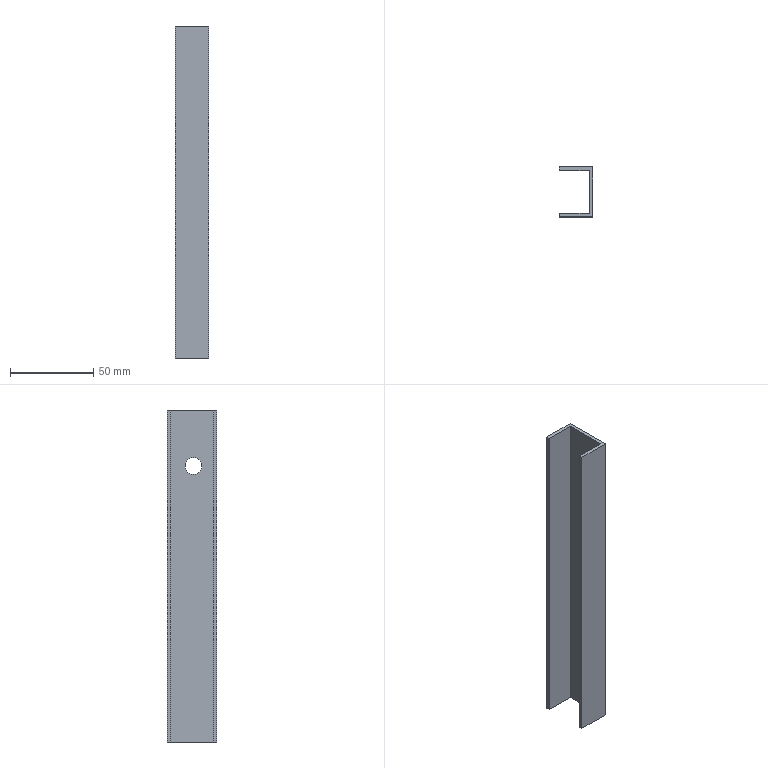Component | SolidWorks | Copy_of_Part3-10 | 1 solid | 12 faces | box 20 x 30 x 200 mm | volume 26243 mm3 | plane 10 | cylinder 2 | commonest cylinder face diameters 10 x2
build123d program:
from build123d import *

# Parameters (mm, degrees)
EXTRUDE_THIN1_DEPTH  = 200
SKETCH3_R            = 5
CUT_EXTRUDE1_2_DEPTH = 10


with BuildPart() as part:
    # Sketch1_2 → Extrude-Thin1 (new body)
    with BuildSketch(Plane.XY):
        Polygon((-20, 15.876), (0, 15.876), (0, -14.124), (-20, -14.124), (-20, -12.124), (-2, -12.124), (-2, 13.876), (-20, 13.876), align=None)
    extrude(amount=EXTRUDE_THIN1_DEPTH)

    # Sketch3 → Cut-Extrude1_2 (cut)
    with BuildSketch(Plane(origin=(0, 0, 0), x_dir=(0, 0, -1), z_dir=(1, 0, 0))):
        with Locations((-166.281, 0)):
            Circle(SKETCH3_R)
    extrude(amount=-CUT_EXTRUDE1_2_DEPTH, mode=Mode.SUBTRACT)


solid = part.part

# Placed as in the assembly
solid = solid.moved(Location((152, 214.124, -1266.092), (0, 0, 0)))
STEP:
#1=COLOUR_RGB('',0.7922,0.8196,0.9333);
#2=FILL_AREA_STYLE_COLOUR('',#1);
#3=FILL_AREA_STYLE('',(#2));
#4=SURFACE_STYLE_FILL_AREA(#3);
#5=SURFACE_SIDE_STYLE('',(#4));
#6=SURFACE_STYLE_USAGE(.BOTH.,#5);
#7=PRESENTATION_STYLE_ASSIGNMENT((#6));
#8=CARTESIAN_POINT('',(5.906,8.43,-43.103));
#9=VERTEX_POINT('',#8);
#10=CARTESIAN_POINT('',(5.906,8.43,-43.496));
#11=VERTEX_POINT('',#10);
#12=CARTESIAN_POINT('',(5.906,8.43,-43.3));
#13=DIRECTION('',(1.,0.,0.));
#14=DIRECTION('',(0.,0.,-1.));
#15=AXIS2_PLACEMENT_3D('',#12,#13,#14);
#16=CIRCLE('',#15,0.1969);
#17=EDGE_CURVE('',#9,#11,#16,.T.);
#18=ORIENTED_EDGE('',*,*,#17,.F.);
#19=CARTESIAN_POINT('',(5.984,8.43,-43.103));
#20=VERTEX_POINT('',#19);
#21=CARTESIAN_POINT('',(5.591,8.43,-43.103));
#22=DIRECTION('',(1.,0.,0.));
#23=VECTOR('',#22,39.37);
#24=LINE('',#21,#23);
#25=EDGE_CURVE('',#9,#20,#24,.T.);
#26=ORIENTED_EDGE('',*,*,#25,.T.);
#27=CARTESIAN_POINT('',(5.984,8.43,-43.496));
#28=VERTEX_POINT('',#27);
#29=CARTESIAN_POINT('',(5.984,8.43,-43.3));
#30=DIRECTION('',(1.,0.,0.));
#31=DIRECTION('',(0.,0.,-1.));
#32=AXIS2_PLACEMENT_3D('',#29,#30,#31);
#33=CIRCLE('',#32,0.1969);
#34=EDGE_CURVE('',#20,#28,#33,.T.);
#35=ORIENTED_EDGE('',*,*,#34,.T.);
#36=CARTESIAN_POINT('',(5.591,8.43,-43.496));
#37=DIRECTION('',(1.,0.,0.));
#38=VECTOR('',#37,39.37);
#39=LINE('',#36,#38);
#40=EDGE_CURVE('',#11,#28,#39,.T.);
#41=ORIENTED_EDGE('',*,*,#40,.F.);
#42=EDGE_LOOP('',(#18,#26,#35,#41));
#43=FACE_OUTER_BOUND('',#42,.T.);
#44=CARTESIAN_POINT('',(5.591,8.43,-43.3));
#45=DIRECTION('',(1.,0.,0.));
#46=DIRECTION('',(0.,0.,-1.));
#47=AXIS2_PLACEMENT_3D('',#44,#45,#46);
#48=CYLINDRICAL_SURFACE('',#47,0.1969);
#49=ADVANCED_FACE('',(#43),#48,.F.);
#50=CARTESIAN_POINT('',(5.906,7.953,-49.846));
#51=VERTEX_POINT('',#50);
#52=CARTESIAN_POINT('',(5.197,7.953,-49.846));
#53=VERTEX_POINT('',#52);
#54=CARTESIAN_POINT('',(5.984,7.953,-49.846));
#55=DIRECTION('',(-1.,-0.,0.));
#56=VECTOR('',#55,39.37);
#57=LINE('',#54,#56);
#58=EDGE_CURVE('',#51,#53,#57,.T.);
#59=ORIENTED_EDGE('',*,*,#58,.T.);
#60=CARTESIAN_POINT('',(5.197,7.953,-41.972));
#61=VERTEX_POINT('',#60);
#62=CARTESIAN_POINT('',(5.197,7.953,-41.972));
#63=DIRECTION('',(0.,0.,-1.));
#64=VECTOR('',#63,39.37);
#65=LINE('',#62,#64);
#66=EDGE_CURVE('',#61,#53,#65,.T.);
#67=ORIENTED_EDGE('',*,*,#66,.F.);
#68=CARTESIAN_POINT('',(5.906,7.953,-41.972));
#69=VERTEX_POINT('',#68);
#70=CARTESIAN_POINT('',(5.984,7.953,-41.972));
#71=DIRECTION('',(-1.,-0.,0.));
#72=VECTOR('',#71,39.37);
#73=LINE('',#70,#72);
#74=EDGE_CURVE('',#69,#61,#73,.T.);
#75=ORIENTED_EDGE('',*,*,#74,.F.);
#76=CARTESIAN_POINT('',(5.906,7.953,-41.972));
#77=DIRECTION('',(0.,0.,-1.));
#78=VECTOR('',#77,39.37);
#79=LINE('',#76,#78);
#80=EDGE_CURVE('',#69,#51,#79,.T.);
#81=ORIENTED_EDGE('',*,*,#80,.T.);
#82=EDGE_LOOP('',(#59,#67,#75,#81));
#83=FACE_OUTER_BOUND('',#82,.T.);
#84=CARTESIAN_POINT('',(5.984,7.953,-41.972));
#85=DIRECTION('',(0.,-1.,0.));
#86=DIRECTION('',(1.,0.,0.));
#87=AXIS2_PLACEMENT_3D('',#84,#85,#86);
#88=PLANE('',#87);
#89=ADVANCED_FACE('',(#83),#88,.F.);
#90=CARTESIAN_POINT('',(5.197,7.874,-49.846));
#91=VERTEX_POINT('',#90);
#92=CARTESIAN_POINT('',(5.197,7.874,-49.846));
#93=DIRECTION('',(0.,1.,0.));
#94=VECTOR('',#93,39.37);
#95=LINE('',#92,#94);
#96=EDGE_CURVE('',#91,#53,#95,.T.);
#97=ORIENTED_EDGE('',*,*,#96,.F.);
#98=CARTESIAN_POINT('',(5.197,7.874,-41.972));
#99=VERTEX_POINT('',#98);
#100=CARTESIAN_POINT('',(5.197,7.874,-41.972));
#101=DIRECTION('',(0.,0.,-1.));
#102=VECTOR('',#101,39.37);
#103=LINE('',#100,#102);
#104=EDGE_CURVE('',#99,#91,#103,.T.);
#105=ORIENTED_EDGE('',*,*,#104,.F.);
#106=CARTESIAN_POINT('',(5.197,7.874,-41.972));
#107=DIRECTION('',(0.,1.,0.));
#108=VECTOR('',#107,39.37);
#109=LINE('',#106,#108);
#110=EDGE_CURVE('',#99,#61,#109,.T.);
#111=ORIENTED_EDGE('',*,*,#110,.T.);
#112=ORIENTED_EDGE('',*,*,#66,.T.);
#113=EDGE_LOOP('',(#97,#105,#111,#112));
#114=FACE_OUTER_BOUND('',#113,.T.);
#115=CARTESIAN_POINT('',(5.197,7.874,-41.972));
#116=DIRECTION('',(-1.,0.,0.));
#117=DIRECTION('',(0.,0.,1.));
#118=AXIS2_PLACEMENT_3D('',#115,#116,#117);
#119=PLANE('',#118);
#120=ADVANCED_FACE('',(#114),#119,.T.);
#121=CARTESIAN_POINT('',(5.984,7.874,-49.846));
#122=VERTEX_POINT('',#121);
#123=CARTESIAN_POINT('',(5.984,7.874,-49.846));
#124=DIRECTION('',(-1.,-0.,0.));
#125=VECTOR('',#124,39.37);
#126=LINE('',#123,#125);
#127=EDGE_CURVE('',#122,#91,#126,.T.);
#128=ORIENTED_EDGE('',*,*,#127,.F.);
#129=CARTESIAN_POINT('',(5.984,7.874,-41.972));
#130=VERTEX_POINT('',#129);
#131=CARTESIAN_POINT('',(5.984,7.874,-41.972));
#132=DIRECTION('',(0.,0.,-1.));
#133=VECTOR('',#132,39.37);
#134=LINE('',#131,#133);
#135=EDGE_CURVE('',#130,#122,#134,.T.);
#136=ORIENTED_EDGE('',*,*,#135,.F.);
#137=CARTESIAN_POINT('',(5.984,7.874,-41.972));
#138=DIRECTION('',(-1.,-0.,0.));
#139=VECTOR('',#138,39.37);
#140=LINE('',#137,#139);
#141=EDGE_CURVE('',#130,#99,#140,.T.);
#142=ORIENTED_EDGE('',*,*,#141,.T.);
#143=ORIENTED_EDGE('',*,*,#104,.T.);
#144=EDGE_LOOP('',(#128,#136,#142,#143));
#145=FACE_OUTER_BOUND('',#144,.T.);
#146=CARTESIAN_POINT('',(5.984,7.874,-41.972));
#147=DIRECTION('',(0.,-1.,0.));
#148=DIRECTION('',(1.,0.,0.));
#149=AXIS2_PLACEMENT_3D('',#146,#147,#148);
#150=PLANE('',#149);
#151=ADVANCED_FACE('',(#145),#150,.T.);
#152=CARTESIAN_POINT('',(5.984,8.43,-43.3));
#153=DIRECTION('',(1.,0.,0.));
#154=DIRECTION('',(0.,0.,-1.));
#155=AXIS2_PLACEMENT_3D('',#152,#153,#154);
#156=CIRCLE('',#155,0.1969);
#157=EDGE_CURVE('',#28,#20,#156,.T.);
#158=ORIENTED_EDGE('',*,*,#157,.F.);
#159=ORIENTED_EDGE('',*,*,#34,.F.);
#160=EDGE_LOOP('',(#158,#159));
#161=FACE_BOUND('',#160,.T.);
#162=CARTESIAN_POINT('',(5.984,9.055,-49.846));
#163=VERTEX_POINT('',#162);
#164=CARTESIAN_POINT('',(5.984,7.874,-49.846));
#165=DIRECTION('',(0.,-1.,0.));
#166=VECTOR('',#165,39.37);
#167=LINE('',#164,#166);
#168=EDGE_CURVE('',#163,#122,#167,.T.);
#169=ORIENTED_EDGE('',*,*,#168,.F.);
#170=CARTESIAN_POINT('',(5.984,9.055,-41.972));
#171=VERTEX_POINT('',#170);
#172=CARTESIAN_POINT('',(5.984,9.055,-41.972));
#173=DIRECTION('',(0.,0.,-1.));
#174=VECTOR('',#173,39.37);
#175=LINE('',#172,#174);
#176=EDGE_CURVE('',#171,#163,#175,.T.);
#177=ORIENTED_EDGE('',*,*,#176,.F.);
#178=CARTESIAN_POINT('',(5.984,7.874,-41.972));
#179=DIRECTION('',(0.,-1.,0.));
#180=VECTOR('',#179,39.37);
#181=LINE('',#178,#180);
#182=EDGE_CURVE('',#171,#130,#181,.T.);
#183=ORIENTED_EDGE('',*,*,#182,.T.);
#184=ORIENTED_EDGE('',*,*,#135,.T.);
#185=EDGE_LOOP('',(#169,#177,#183,#184));
#186=FACE_OUTER_BOUND('',#185,.T.);
#187=CARTESIAN_POINT('',(5.984,7.874,-41.972));
#188=DIRECTION('',(1.,0.,0.));
#189=DIRECTION('',(0.,0.,-1.));
#190=AXIS2_PLACEMENT_3D('',#187,#188,#189);
#191=PLANE('',#190);
#192=ADVANCED_FACE('',(#161,#186),#191,.T.);
#193=CARTESIAN_POINT('',(5.197,9.055,-49.846));
#194=VERTEX_POINT('',#193);
#195=CARTESIAN_POINT('',(5.984,9.055,-49.846));
#196=DIRECTION('',(1.,0.,0.));
#197=VECTOR('',#196,39.37);
#198=LINE('',#195,#197);
#199=EDGE_CURVE('',#194,#163,#198,.T.);
#200=ORIENTED_EDGE('',*,*,#199,.F.);
#201=CARTESIAN_POINT('',(5.197,9.055,-41.972));
#202=VERTEX_POINT('',#201);
#203=CARTESIAN_POINT('',(5.197,9.055,-41.972));
#204=DIRECTION('',(0.,0.,-1.));
#205=VECTOR('',#204,39.37);
#206=LINE('',#203,#205);
#207=EDGE_CURVE('',#202,#194,#206,.T.);
#208=ORIENTED_EDGE('',*,*,#207,.F.);
#209=CARTESIAN_POINT('',(5.984,9.055,-41.972));
#210=DIRECTION('',(1.,0.,0.));
#211=VECTOR('',#210,39.37);
#212=LINE('',#209,#211);
#213=EDGE_CURVE('',#202,#171,#212,.T.);
#214=ORIENTED_EDGE('',*,*,#213,.T.);
#215=ORIENTED_EDGE('',*,*,#176,.T.);
#216=EDGE_LOOP('',(#200,#208,#214,#215));
#217=FACE_OUTER_BOUND('',#216,.T.);
#218=CARTESIAN_POINT('',(5.984,9.055,-41.972));
#219=DIRECTION('',(0.,1.,0.));
#220=DIRECTION('',(0.,0.,1.));
#221=AXIS2_PLACEMENT_3D('',#218,#219,#220);
#222=PLANE('',#221);
#223=ADVANCED_FACE('',(#217),#222,.T.);
#224=CARTESIAN_POINT('',(5.197,8.976,-49.846));
#225=VERTEX_POINT('',#224);
#226=CARTESIAN_POINT('',(5.197,8.976,-49.846));
#227=DIRECTION('',(0.,1.,0.));
#228=VECTOR('',#227,39.37);
#229=LINE('',#226,#228);
#230=EDGE_CURVE('',#225,#194,#229,.T.);
#231=ORIENTED_EDGE('',*,*,#230,.F.);
#232=CARTESIAN_POINT('',(5.197,8.976,-41.972));
#233=VERTEX_POINT('',#232);
#234=CARTESIAN_POINT('',(5.197,8.976,-41.972));
#235=DIRECTION('',(0.,0.,-1.));
#236=VECTOR('',#235,39.37);
#237=LINE('',#234,#236);
#238=EDGE_CURVE('',#233,#225,#237,.T.);
#239=ORIENTED_EDGE('',*,*,#238,.F.);
#240=CARTESIAN_POINT('',(5.197,8.976,-41.972));
#241=DIRECTION('',(0.,1.,0.));
#242=VECTOR('',#241,39.37);
#243=LINE('',#240,#242);
#244=EDGE_CURVE('',#233,#202,#243,.T.);
#245=ORIENTED_EDGE('',*,*,#244,.T.);
#246=ORIENTED_EDGE('',*,*,#207,.T.);
#247=EDGE_LOOP('',(#231,#239,#245,#246));
#248=FACE_OUTER_BOUND('',#247,.T.);
#249=CARTESIAN_POINT('',(5.197,8.976,-41.972));
#250=DIRECTION('',(-1.,0.,0.));
#251=DIRECTION('',(0.,0.,1.));
#252=AXIS2_PLACEMENT_3D('',#249,#250,#251);
#253=PLANE('',#252);
#254=ADVANCED_FACE('',(#248),#253,.T.);
#255=CARTESIAN_POINT('',(5.906,8.976,-49.846));
#256=VERTEX_POINT('',#255);
#257=CARTESIAN_POINT('',(5.984,8.976,-49.846));
#258=DIRECTION('',(1.,0.,0.));
#259=VECTOR('',#258,39.37);
#260=LINE('',#257,#259);
#261=EDGE_CURVE('',#225,#256,#260,.T.);
#262=ORIENTED_EDGE('',*,*,#261,.T.);
#263=CARTESIAN_POINT('',(5.906,8.976,-41.972));
#264=VERTEX_POINT('',#263);
#265=CARTESIAN_POINT('',(5.906,8.976,-41.972));
#266=DIRECTION('',(0.,0.,-1.));
#267=VECTOR('',#266,39.37);
#268=LINE('',#265,#267);
#269=EDGE_CURVE('',#264,#256,#268,.T.);
#270=ORIENTED_EDGE('',*,*,#269,.F.);
#271=CARTESIAN_POINT('',(5.984,8.976,-41.972));
#272=DIRECTION('',(1.,0.,0.));
#273=VECTOR('',#272,39.37);
#274=LINE('',#271,#273);
#275=EDGE_CURVE('',#233,#264,#274,.T.);
#276=ORIENTED_EDGE('',*,*,#275,.F.);
#277=ORIENTED_EDGE('',*,*,#238,.T.);
#278=EDGE_LOOP('',(#262,#270,#276,#277));
#279=FACE_OUTER_BOUND('',#278,.T.);
#280=CARTESIAN_POINT('',(5.984,8.976,-41.972));
#281=DIRECTION('',(0.,1.,0.));
#282=DIRECTION('',(0.,0.,1.));
#283=AXIS2_PLACEMENT_3D('',#280,#281,#282);
#284=PLANE('',#283);
#285=ADVANCED_FACE('',(#279),#284,.F.);
#286=CARTESIAN_POINT('',(5.906,8.43,-43.3));
#287=DIRECTION('',(1.,0.,0.));
#288=DIRECTION('',(0.,0.,-1.));
#289=AXIS2_PLACEMENT_3D('',#286,#287,#288);
#290=CIRCLE('',#289,0.1969);
#291=EDGE_CURVE('',#11,#9,#290,.T.);
#292=ORIENTED_EDGE('',*,*,#291,.T.);
#293=ORIENTED_EDGE('',*,*,#17,.T.);
#294=EDGE_LOOP('',(#292,#293));
#295=FACE_BOUND('',#294,.T.);
#296=CARTESIAN_POINT('',(5.906,7.874,-49.846));
#297=DIRECTION('',(0.,-1.,0.));
#298=VECTOR('',#297,39.37);
#299=LINE('',#296,#298);
#300=EDGE_CURVE('',#256,#51,#299,.T.);
#301=ORIENTED_EDGE('',*,*,#300,.T.);
#302=ORIENTED_EDGE('',*,*,#80,.F.);
#303=CARTESIAN_POINT('',(5.906,7.874,-41.972));
#304=DIRECTION('',(0.,-1.,0.));
#305=VECTOR('',#304,39.37);
#306=LINE('',#303,#305);
#307=EDGE_CURVE('',#264,#69,#306,.T.);
#308=ORIENTED_EDGE('',*,*,#307,.F.);
#309=ORIENTED_EDGE('',*,*,#269,.T.);
#310=EDGE_LOOP('',(#301,#302,#308,#309));
#311=FACE_OUTER_BOUND('',#310,.T.);
#312=CARTESIAN_POINT('',(5.906,7.874,-41.972));
#313=DIRECTION('',(1.,0.,0.));
#314=DIRECTION('',(0.,0.,-1.));
#315=AXIS2_PLACEMENT_3D('',#312,#313,#314);
#316=PLANE('',#315);
#317=ADVANCED_FACE('',(#295,#311),#316,.F.);
#318=ORIENTED_EDGE('',*,*,#74,.T.);
#319=ORIENTED_EDGE('',*,*,#110,.F.);
#320=ORIENTED_EDGE('',*,*,#141,.F.);
#321=ORIENTED_EDGE('',*,*,#182,.F.);
#322=ORIENTED_EDGE('',*,*,#213,.F.);
#323=ORIENTED_EDGE('',*,*,#244,.F.);
#324=ORIENTED_EDGE('',*,*,#275,.T.);
#325=ORIENTED_EDGE('',*,*,#307,.T.);
#326=EDGE_LOOP('',(#318,#319,#320,#321,#322,#323,#324,#325));
#327=FACE_OUTER_BOUND('',#326,.T.);
#328=CARTESIAN_POINT('',(5.984,8.43,-41.972));
#329=DIRECTION('',(0.,0.,-1.));
#330=DIRECTION('',(-1.,0.,0.));
#331=AXIS2_PLACEMENT_3D('',#328,#329,#330);
#332=PLANE('',#331);
#333=ADVANCED_FACE('',(#327),#332,.F.);
#334=ORIENTED_EDGE('',*,*,#58,.F.);
#335=ORIENTED_EDGE('',*,*,#300,.F.);
#336=ORIENTED_EDGE('',*,*,#261,.F.);
#337=ORIENTED_EDGE('',*,*,#230,.T.);
#338=ORIENTED_EDGE('',*,*,#199,.T.);
#339=ORIENTED_EDGE('',*,*,#168,.T.);
#340=ORIENTED_EDGE('',*,*,#127,.T.);
#341=ORIENTED_EDGE('',*,*,#96,.T.);
#342=EDGE_LOOP('',(#334,#335,#336,#337,#338,#339,#340,#341));
#343=FACE_OUTER_BOUND('',#342,.T.);
#344=CARTESIAN_POINT('',(5.984,8.43,-49.846));
#345=DIRECTION('',(0.,0.,-1.));
#346=DIRECTION('',(-1.,0.,0.));
#347=AXIS2_PLACEMENT_3D('',#344,#345,#346);
#348=PLANE('',#347);
#349=ADVANCED_FACE('',(#343),#348,.T.);
#350=ORIENTED_EDGE('',*,*,#25,.F.);
#351=ORIENTED_EDGE('',*,*,#291,.F.);
#352=ORIENTED_EDGE('',*,*,#40,.T.);
#353=ORIENTED_EDGE('',*,*,#157,.T.);
#354=EDGE_LOOP('',(#350,#351,#352,#353));
#355=FACE_OUTER_BOUND('',#354,.T.);
#356=CARTESIAN_POINT('',(5.591,8.43,-43.3));
#357=DIRECTION('',(1.,0.,0.));
#358=DIRECTION('',(0.,0.,-1.));
#359=AXIS2_PLACEMENT_3D('',#356,#357,#358);
#360=CYLINDRICAL_SURFACE('',#359,0.1969);
#361=ADVANCED_FACE('',(#355),#360,.F.);
#362=CLOSED_SHELL('',(#49,#89,#120,#151,#192,#223,#254,#285,#317,#333,#349,#361));
#363=MANIFOLD_SOLID_BREP('',#362);
#364=STYLED_ITEM('',(#7),#363);
#365=PRESENTATION_LAYER_ASSIGNMENT('','',(#364));
#366=CARTESIAN_POINT('',(0.,0.,0.));
#367=DIRECTION('',(0.,0.,1.));
#368=DIRECTION('',(1.,0.,0.));
#369=AXIS2_PLACEMENT_3D('',#366,#367,#368);
#370=(LENGTH_UNIT()NAMED_UNIT(*)SI_UNIT($,.METRE.));
#371=LENGTH_MEASURE_WITH_UNIT(LENGTH_MEASURE(0.0254),#370);
#372=DIMENSIONAL_EXPONENTS(1.,0.,0.,0.,0.,0.,0.);
#373=(CONVERSION_BASED_UNIT('',#371)LENGTH_UNIT()NAMED_UNIT(#372));
#374=UNCERTAINTY_MEASURE_WITH_UNIT(LENGTH_MEASURE(0.00001),#373,'','');
#375=(NAMED_UNIT(*)PLANE_ANGLE_UNIT()SI_UNIT($,.RADIAN.));
#376=(NAMED_UNIT(*)SI_UNIT($,.STERADIAN.)SOLID_ANGLE_UNIT());
#377=(GEOMETRIC_REPRESENTATION_CONTEXT(3)GLOBAL_UNCERTAINTY_ASSIGNED_CONTEXT((#374))GLOBAL_UNIT_ASSIGNED_CONTEXT((#373,#375,#376))REPRESENTATION_CONTEXT('',''));
#378=ADVANCED_BREP_SHAPE_REPRESENTATION('',(#363,#369),#377);
#379=(LENGTH_UNIT()NAMED_UNIT(*)SI_UNIT($,.METRE.));
#380=LENGTH_MEASURE_WITH_UNIT(LENGTH_MEASURE(0.0254),#379);
#381=DIMENSIONAL_EXPONENTS(1.,0.,0.,0.,0.,0.,0.);
#382=(CONVERSION_BASED_UNIT('',#380)LENGTH_UNIT()NAMED_UNIT(#381));
#383=UNCERTAINTY_MEASURE_WITH_UNIT(LENGTH_MEASURE(0.00001),#382,'','');
#384=(NAMED_UNIT(*)PLANE_ANGLE_UNIT()SI_UNIT($,.RADIAN.));
#385=(NAMED_UNIT(*)SI_UNIT($,.STERADIAN.)SOLID_ANGLE_UNIT());
#386=(GEOMETRIC_REPRESENTATION_CONTEXT(3)GLOBAL_UNCERTAINTY_ASSIGNED_CONTEXT((#383))GLOBAL_UNIT_ASSIGNED_CONTEXT((#382,#384,#385))REPRESENTATION_CONTEXT('',''));
#387=MECHANICAL_DESIGN_GEOMETRIC_PRESENTATION_REPRESENTATION('',(#364),#386);